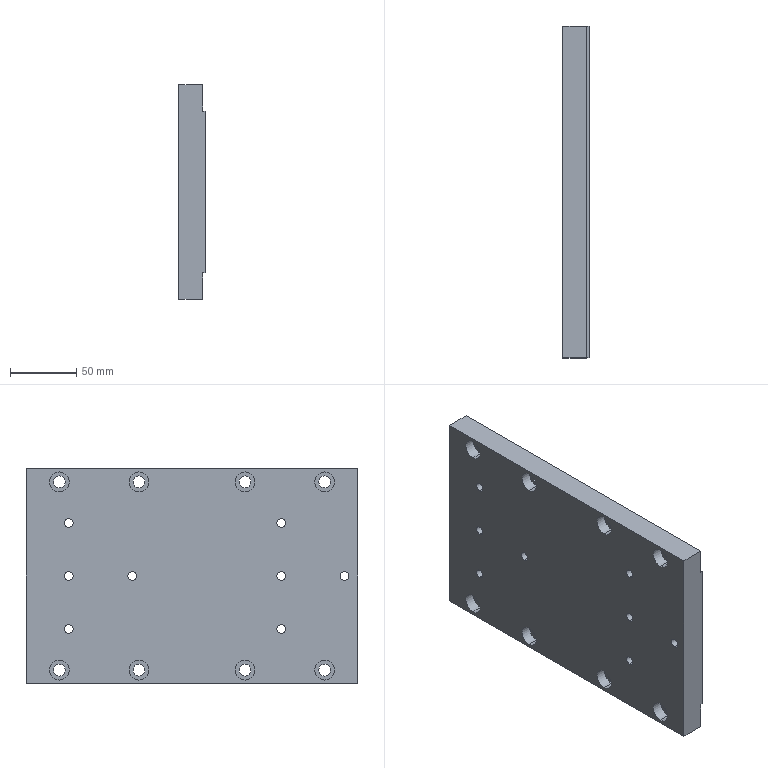Component | SolidWorks | F8-1 | 1 solid | 90 faces | box 20 x 250 x 162 mm | volume 765208 mm3 | cylinder 64 | plane 26 | commonest cylinder face diameters 15 x16 9 x16 11 x16 6.6 x16
build123d program:
from build123d import *

# Parameters (mm, degrees)
SKETCH1_W                                       = 162
SKETCH1_H                                       = 270
BOSS_EXTRUDE1_DEPTH                             = 20
SKETCH3_W                                       = 162
SKETCH3_H                                       = 20
CUT_EXTRUDE1_DEPTH                              = 20
M6_HEX_SOCKET_HEAD_CAP_SCREW_CBORE1_D           = 6.6
M6_HEX_SOCKET_HEAD_CAP_SCREW_CBORE1_CBORE_D     = 11
M6_HEX_SOCKET_HEAD_CAP_SCREW_CBORE1_CBORE_DEPTH = 6
SKETCH19_W                                      = 20
SKETCH19_H                                      = 2
CUT_EXTRUDE7_DEPTH                              = 286.778
M8_HEX_SOCKET_HEAD_CAP_SCREW_CBORE1_D           = 9
M8_HEX_SOCKET_HEAD_CAP_SCREW_CBORE1_CBORE_D     = 15
M8_HEX_SOCKET_HEAD_CAP_SCREW_CBORE1_CBORE_DEPTH = 8


with BuildPart() as part:
    # Sketch1 → Boss-Extrude1 (new body)
    with BuildSketch(Plane.XY):
        with Locations((56, 578)):
            Rectangle(SKETCH1_W, SKETCH1_H)
    extrude(amount=BOSS_EXTRUDE1_DEPTH)

    # Sketch3 → Cut-Extrude1 (cut)
    with BuildSketch(Plane.XZ.offset(-443)):
        with Locations((56, 10)):
            Rectangle(SKETCH3_W, SKETCH3_H)
    extrude(amount=-CUT_EXTRUDE1_DEPTH, mode=Mode.SUBTRACT)

    # M6 Hex Socket Head Cap Screw CBORE1 (through all)
    with Locations(Plane.XY.offset(20)):
        with Locations((56, 473), (96, 520.8), (56, 520.8), (16, 520.8), (16, 680.8), (56, 680.8), (96, 680.8), (56, 633)):
            CounterBoreHole(M6_HEX_SOCKET_HEAD_CAP_SCREW_CBORE1_D / 2, M6_HEX_SOCKET_HEAD_CAP_SCREW_CBORE1_CBORE_D / 2, M6_HEX_SOCKET_HEAD_CAP_SCREW_CBORE1_CBORE_DEPTH)

    # Sketch19 → Cut-Extrude7 (cut, through all)
    with BuildSketch(Plane.XZ.offset(-463)):
        with Locations((-15, 19)):
            Rectangle(SKETCH19_W, SKETCH19_H)
        with Locations((127, 19)):
            Rectangle(SKETCH19_W, SKETCH19_H)
    extrude(amount=-CUT_EXTRUDE7_DEPTH, mode=Mode.SUBTRACT)

    # M8 Hex Socket Head Cap Screw CBORE1 (through all)
    with Locations(Plane(origin=(0, 0, 0), x_dir=(-1, 0, 0), z_dir=(0, 0, -1))):
        with Locations((15, 688), (15, 628), (15, 488), (15, 548), (-127, 688), (-127, 628), (-127, 548), (-127, 488)):
            CounterBoreHole(M8_HEX_SOCKET_HEAD_CAP_SCREW_CBORE1_D / 2, M8_HEX_SOCKET_HEAD_CAP_SCREW_CBORE1_CBORE_D / 2, M8_HEX_SOCKET_HEAD_CAP_SCREW_CBORE1_CBORE_DEPTH)


solid = part.part

# Placed as in the assembly
solid = solid.moved(Location((0, -599.721, 0), (0, 90, 0)))